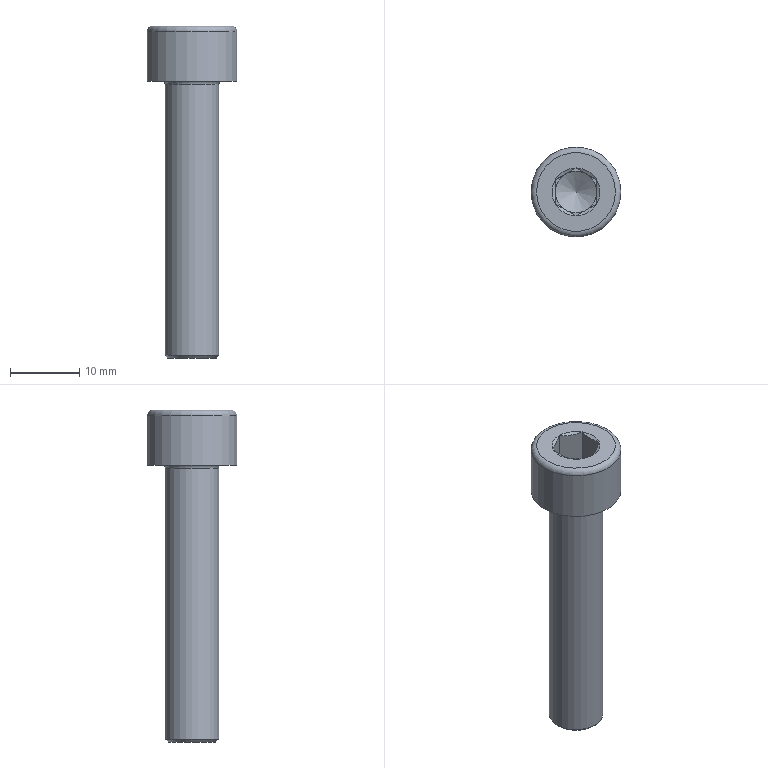Component | NX | GB-T70_1-2000_M8X40 | 1 solid | 27 faces | volume 2783 mm3 | plane 15 | cone 8 | cylinder 2 | torus 2 | commonest cylinder face diameters 7.76 x1 13 x1